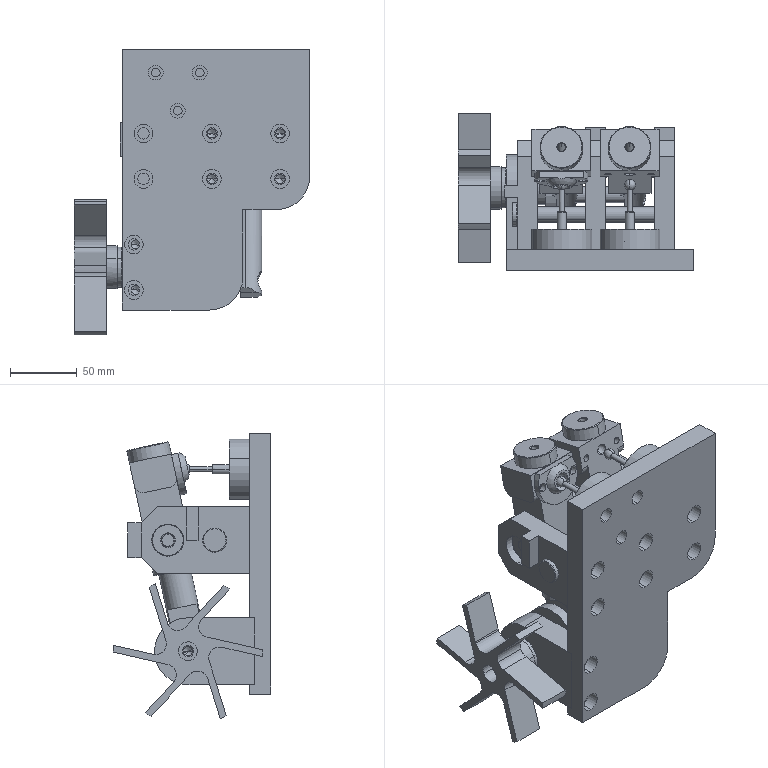Assembly | SolidWorks | mm | 24 component files | 24 solids | 680 faces | box 176.05 x 118 x 213.55 mm | volume 944515 mm3 | cylinder 298 | plane 217 | cone 130 | torus 16 | sphere 15 | spline 4 | commonest cylinder face diameters 12 x45 10 x40 14 x26 5 x24 24 x22 8.5 x18 6.8 x16 6.5 x14
Bill of materials:
BasePlate | 1 |  | Flat plate with a stepped L-like outline: a rectangular notch is cut from one lower corner, and the outer corners at the step are rounded. It has a pattern of about 11 through holes in two sizes.
BearingBlock | 2 |  | Short solid cylinder (disc) with three small holes spaced around the outside edge of one face.
BracketOne | 1 |  | Rectangular block with one semicircular rounded end. A large cross bore goes through near the rounded end, and two small holes are drilled into the opposite flat end face.
BracketThree | 1 |  | Flat plate with one end chamfered at both corners. It has a small and a large through hole on its centerline and a small rectangular tab sticking out from one edge.
BracketTwo | 2 |  | Flat plate that tapers through angled shoulders into a narrower rectangular tab at one end. It has a small and a large through hole on its centerline and two small holes in the opposite end face.
Crank | 1 |  | Irregular curved plate shaped like a cam or lever, with a concave notch. It has a large cylindrical boss on one face, a smaller boss on the other face, and two holes inside annular recessed rings.
Gland | 1 |  | Flange shaped like a circular disc cut flat along one chord. It has two through mounting holes and a central raised dome-like boss containing a recessed elongated socket.
GuidePost | 2 |  | Stepped round pin. A small sphere sits at one end on a thin shaft, followed by a larger-diameter cylindrical section with a rounded, hemispherical far end.
Impeller | 1 |  | Six-armed star or impeller-like part. Straight narrow arms extend from a central hub, which has a small central hole and a short cylindrical boss on one side.
Ornament | 1 |  | Housing-like body with a rectangular main block, cylindrical spigots at both ends (one hollow), a top cylindrical boss with a small central hole, a widened upper section with three holes, and two side-mounted cylindrical pins.
Ornament | 1 |  | Elongated block with a rectangular cross-section and a cylindrical boss at each end. One end has a wider rectangular flange with three holes in a row across it: a larger hole in the middle and a smaller hole on each side. Near the other end, a short cylindrical pin sticks out of each of two opposite side faces. The end boss next to the flange has a small hole in its center. The opposite end boss looks hollow, like an open ring.
Part1 | 1 |  | Plain solid cylindrical rod with flat ends and no visible features.
RetainingRing | 1 |  | Flanged sleeve or bushing: a hollow cylinder with a larger-diameter flange at one end, a central through bore, and chamfered outer edges.
RotationAxis | 1 |  | Stepped, roughly axisymmetric body with a thin raised flange near one end. A short cylindrical section sits on one side of the flange. On the other side is a longer cylindrical body that ends in a narrower end section with a rounded-polygon (rounded square/lobed) cross-section. A small central hole is in that end face.
SwingRod | 2 |  | Solid cylindrical pin. About half its length has full circular section. Part of the remaining length has material cut away, leaving a stepped, partly flat (D-like) section. A small hole goes crosswise through the cut-down part near the end.
TieRod | 1 |  | Long, slender tube-like pin with a thin round head flange at one end and an axial bore.
Washer | 4 |  | Flat annular ring (plain washer-like disc) with a central round hole and small chamfers on the outer edges.
Mates:
1. coincident | BasePlate-1 face at (135.246, 0, 348.671) dir (0, -1, 0) | assembly plane at (0, 0, 0) dir (0, 1, 0)
2. coincident | BasePlate-1 face at (92.128, 12, 330.671) dir (0, 1, 0) | BracketOne-1 face at (90.246, 12, 380.671) dir (0, -1, 0)
3. coincident | BasePlate-1 face at (90.246, 12, 335.303) dir (-1, 0, 0) | BracketOne-1 face at (90.246, 62, 355.671) dir (1, 0, 0)
4. coincident | BasePlate-1 face at (70.246, 12, 330.671) dir (0, 0, 1) | BracketOne-1 face at (90.246, 62, 330.671) dir (0, 0, -1)
5. concentric | RotationAxis-1 face at (96.296, 62, 355.671) dir (1, 0, 0) r 2.5 | Crank-1 face at (113.297, 62, 355.671) dir (-1, 0, 0) r 3.25
6. coincident | RotationAxis-1 face at (96.296, 63.181, 352.339) dir (1, 0, 0) | Crank-1 face at (96.296, 65.332, 356.852) dir (-1, 0, 0)
7. concentric | RotationAxis-1 face at (90.296, 62, 355.671) dir (-1, 0, 0) r 10 | BracketOne-1 face at (90.246, 62, 355.671) dir (-1, 0, 0) r 10
8. width | Crank-1 face at (90.296, 62, 355.671) dir (-1, 0, 0) | RotationAxis-1 face at (70.196, 62, 355.671) dir (1, 0, 0) | BracketOne-1 face at (90.246, 62, 355.671) dir (1, 0, 0) | BracketOne-1 face at (70.246, 62, 355.671) dir (-1, 0, 0)
9. coincident | BasePlate-1 face at (129.546, 12, 413.671) dir (0, 1, 0) | BracketTwo-1 face at (129.546, 12, 413.671) dir (0, -1, 0)
10. coincident | BasePlate-1 face at (129.546, 12, 458.671) dir (1, 0, 0) | BracketTwo-1 face at (129.546, 54.5, 438.671) dir (-1, 0, 0)
11. coincident | BasePlate-1 face at (139.546, 12, 463.671) dir (0, 0, -1) | BracketTwo-1 face at (129.546, 85, 463.671) dir (0, 0, 1)
12. coincident | BasePlate-1 face at (93.546, 12, 463.671) dir (0, 1, 0) | BracketThree-1 face at (93.546, 12, 463.671) dir (0, -1, 0)
13. coincident | BasePlate-1 face at (83.546, 12, 413.671) dir (0, 0, 1) | BracketThree-1 face at (93.546, 85, 413.671) dir (0, 0, -1)
14. coincident | BasePlate-1 face at (93.546, 12, 458.671) dir (-1, 0, 0) | BracketThree-1 face at (93.546, 54.5, 438.671) dir (1, 0, 0)
15. concentric | Ornament-1 face at (111.296, 71.958, 415.207) dir (0, -0.2101, -0.9777) r 12 | SwingRod-1 face at (111.296, 54.736, 335.062) dir (0, 0.2101, 0.9777) r 12
16. concentric | SwingRod-1 face at (117.296, 56.837, 344.838) dir (-1, 0, 0) r 6 | Crank-1 face at (113.296, 56.837, 344.838) dir (-1, 0, 0) r 6
17. coincident | SwingRod-1 face at (107.296, 66.291, 388.834) dir (-1, 0, 0) | Crank-1 face at (107.296, 75.667, 342.51) dir (1, 0, 0)
18. concentric | Impeller-1 face at (34.196, 62, 355.671) dir (1, 0, 0) r 16 | RotationAxis-1 face at (70.196, 62, 355.671) dir (-1, 0, 0) r 15
19. coincident | Impeller-1 face at (59.196, 62.692, 366.419) dir (0, -0.4302, -0.9027) | RotationAxis-1 face at (66.196, 62.692, 366.419) dir (0, 0.4302, 0.9027)
20. coincident | Impeller-1 face at (59.196, 63.89, 350.339) dir (1, 0, 0) | RotationAxis-1 face at (59.196, 56.668, 353.781) dir (-1, 0, 0)
21. concentric | Ornament-1 face at (138.296, 77, 438.671) dir (-1, 0, 0) r 5 | BracketTwo-1 face at (138.546, 77, 438.671) dir (-1, 0, 0) r 13
22. concentric | BasePlate-1 face at (111.546, 12, 491.671) dir (0, 1, 0) r 22.5 | BearingBlock-1 face at (111.546, 31, 491.671) dir (0, -1, 0) r 22.5
23. coincident | BasePlate-1 face at (111.546, 12, 491.671) dir (0, 1, 0) | BearingBlock-1 face at (111.546, 12, 491.671) dir (0, -1, 0)
24. coincident | Ornament-1 face at (111.296, 66.242, 464.764) dir (0, -0.9777, 0.2101) | Gland-1 face at (111.296, 72.071, 491.894) dir (0, 0.9777, -0.2101)
25. concentric | Ornament-1 face at (95.296, 72.071, 491.894) dir (0, -0.9777, 0.2101) r 2.5 | Gland-1 face at (95.296, 72.071, 491.894) dir (0, -0.9777, 0.2101) r 3.25
26. concentric | Ornament-1 face at (127.296, 72.071, 491.894) dir (0, -0.9777, 0.2101) r 2.5 | Gland-1 face at (127.296, 72.071, 491.894) dir (0, -0.9777, 0.2101) r 3.25
27. concentric | BracketTwo-1 face at (178.487, 77, 438.671) dir (-1, 0, 0) r 12 | Washer-1 face at (138.546, 77, 438.671) dir (-1, 0, 0) r 5
28. coincident | BracketTwo-1 edge at (138.546, 77, 438.671) dir (-1, 0, 0) r 12 | Washer-1 face at (138.546, 77, 438.671) dir (1, 0, 0)
29. concentric | SwingRod-1 face at (117.296, 56.837, 344.838) dir (-1, 0, 0) r 6 | RetainingRing-1 face at (120.296, 56.837, 344.838) dir (1, 0, 0) r 6
30. coincident | SwingRod-1 face at (117.296, 56.837, 344.838) dir (1, 0, 0) | RetainingRing-1 face at (117.296, 52.789, 338.524) dir (-1, 0, 0)
31. concentric | BracketThree-1 face at (78.545, 77, 438.671) dir (1, 0, 0) r 12 | Washer-5 face at (88.546, 77, 438.671) dir (-1, 0, 0) r 5
32. coincident | BracketThree-1 edge at (84.546, 77, 438.671) dir (1, 0, 0) r 12 | Washer-5 face at (84.546, 77, 438.671) dir (-1, 0, 0)
33. concentric | BracketThree-1 face at (93.546, 42, 438.671) dir (-1, 0, 0) r 6 | TieRod-1 face at (78.546, 42, 438.671) dir (1, 0, 0) r 6
34. coincident | BracketThree-1 face at (78.546, 54.5, 438.671) dir (-1, 0, 0) | TieRod-1 face at (78.546, 42, 438.671) dir (1, 0, 0)
35. concentric | BearingBlock-1 face at (111.546, 26, 491.671) dir (0, 1, 0) r 18.165 | GuidePost-1 face at (111.546, 68.028, 491.671) dir (0, 1, 0) r 3.5
36. tangent | Ornament-1 face at (111.296, 72.071, 491.894) dir (1, 0, 0) r 4.05 | GuidePost-1 face at (111.546, 64.028, 491.671) dir (1, 0, 0) r 4
37. coincident | RotationAxis-1 face at (96.296, 63.4, 364.42) dir (0, 0.4302, 0.9027) | Crank-1 face at (96.296, 63.4, 364.42) dir (0, -0.4302, -0.9027)